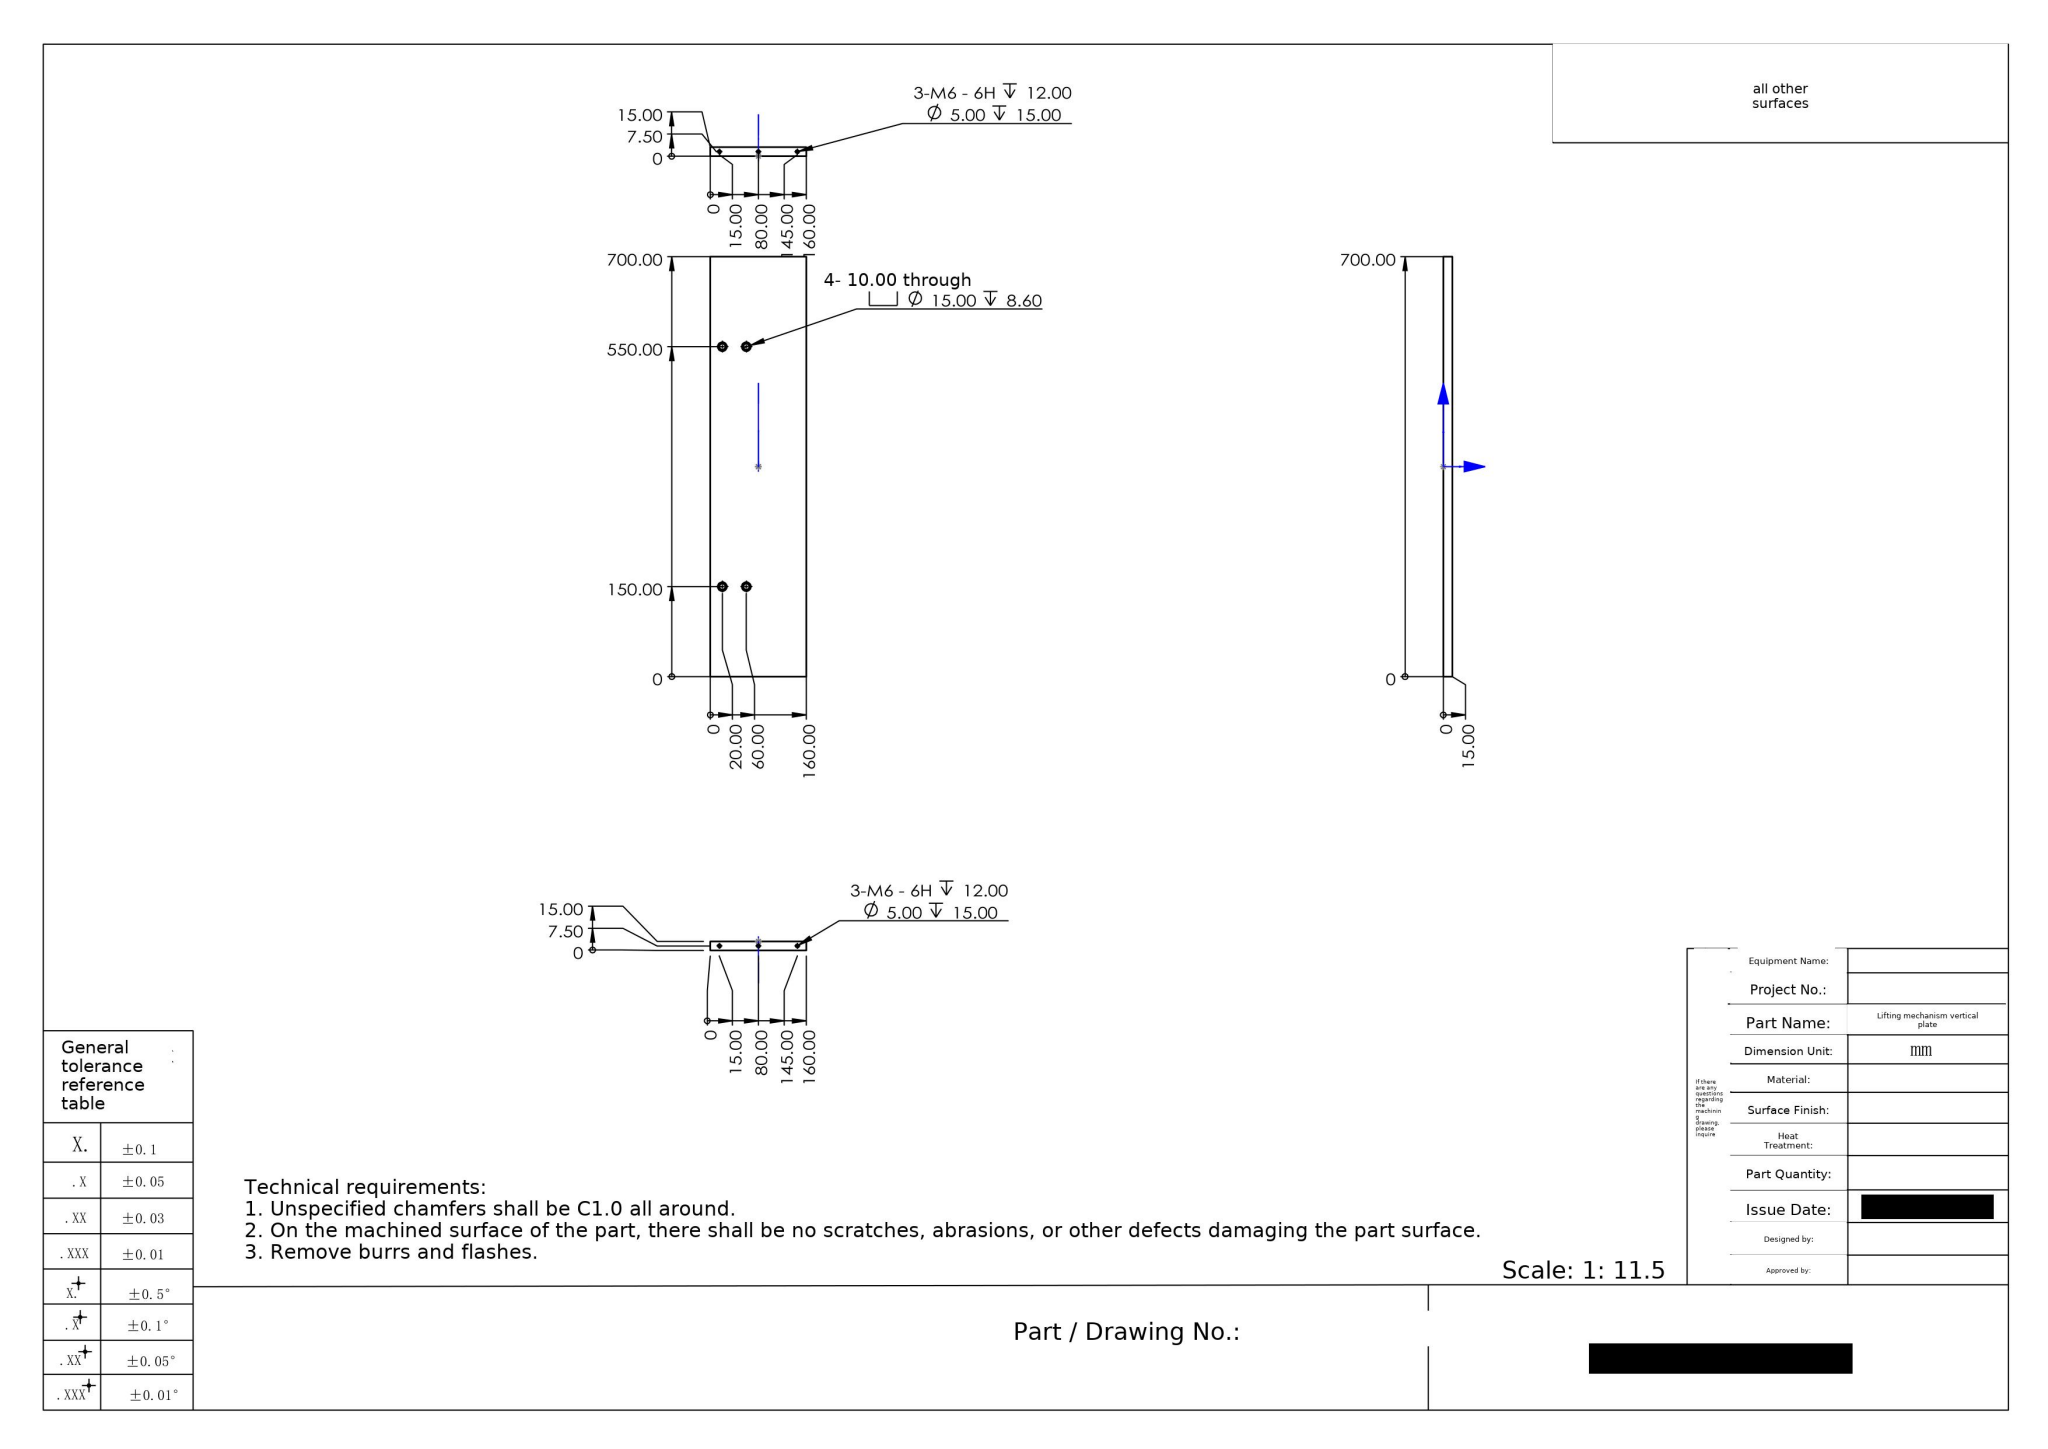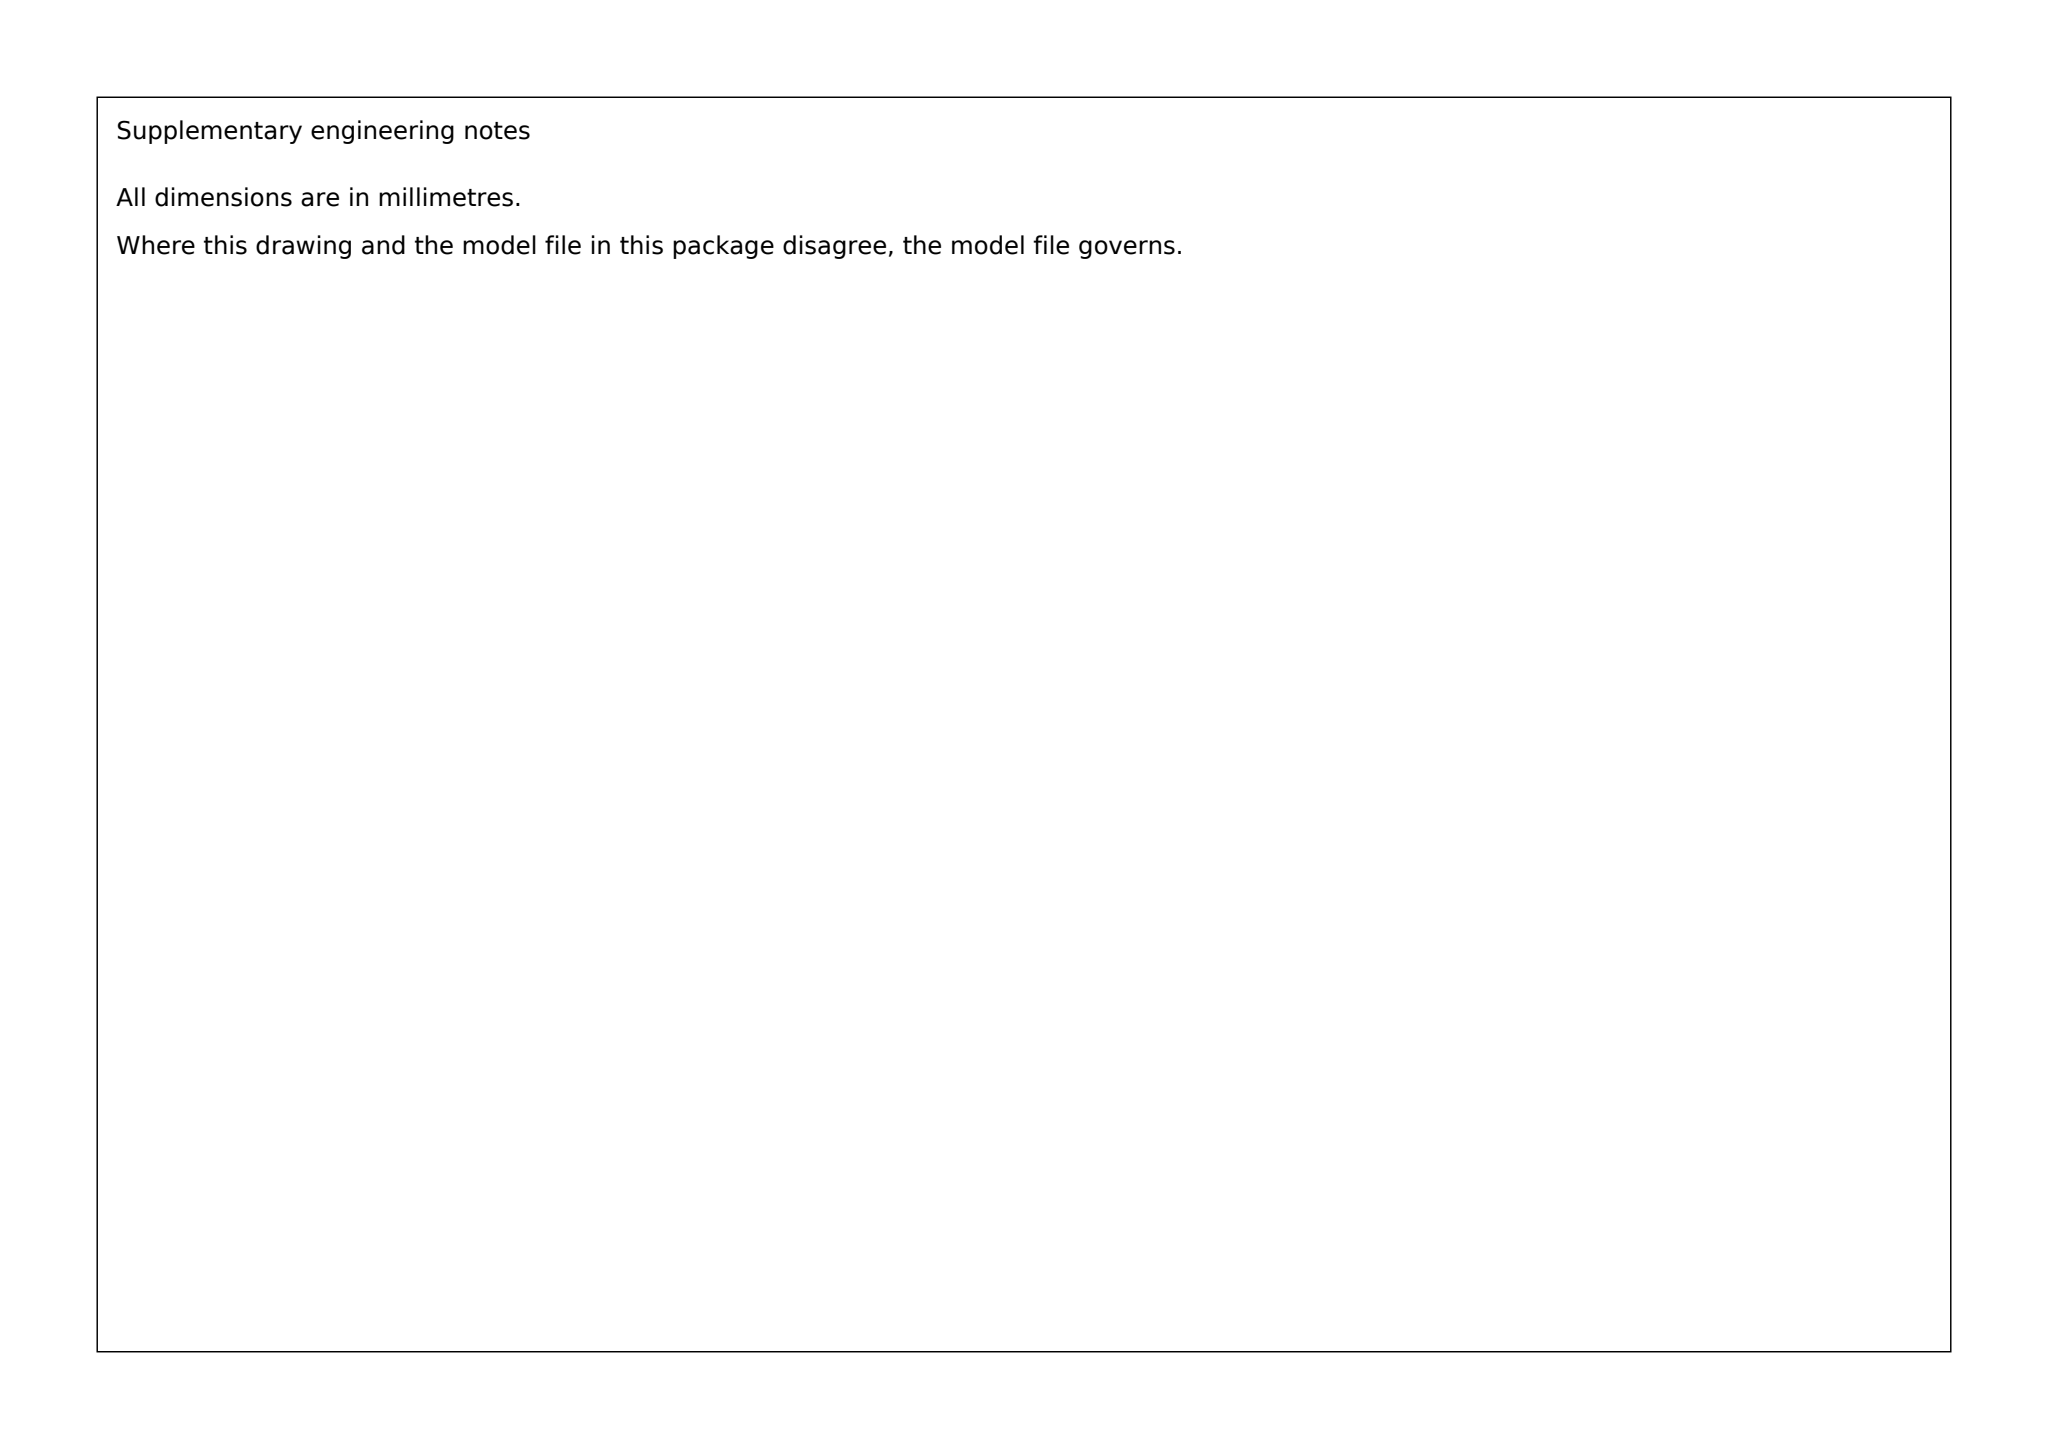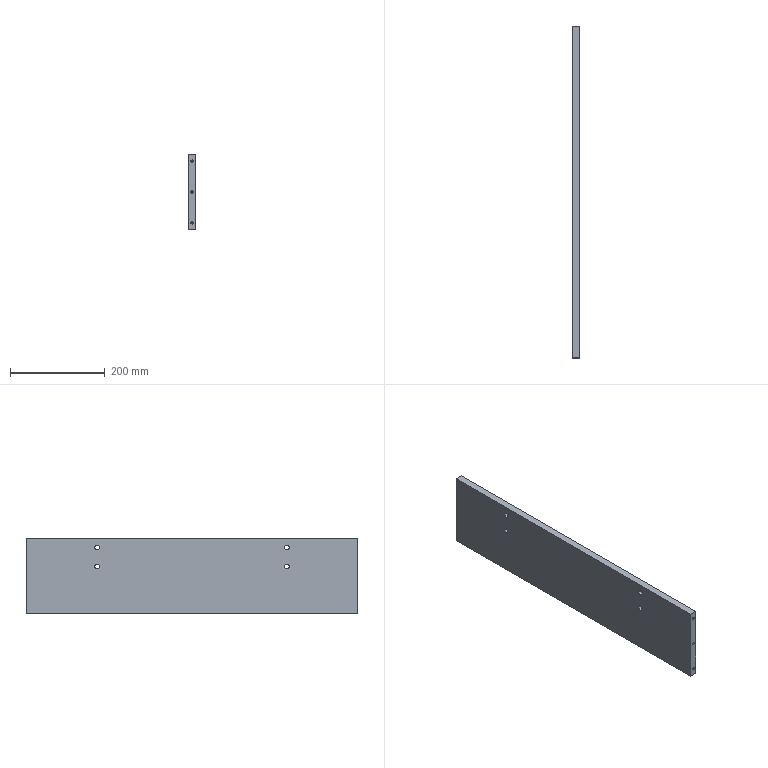Part | SolidWorks | mm | 1 solid | 50 faces | box 15 x 700 x 160 mm | volume 1670084 mm3 | cylinder 28 | cone 12 | plane 10 | commonest cylinder face diameters 5 x12 15 x8 10 x8
build123d program:
from build123d import *

# Parameters (mm, degrees)
SKETCH1_W                                       = 160
SKETCH1_H                                       = 700
BOSS_EXTRUDE1_DEPTH                             = 15
M8_HEX_SOCKET_HEAD_CAP_SCREW_CBORE1_D           = 10
M8_HEX_SOCKET_HEAD_CAP_SCREW_CBORE1_CBORE_D     = 15
M8_HEX_SOCKET_HEAD_CAP_SCREW_CBORE1_CBORE_DEPTH = 8.6
M6_TAPPED_HOLE1_AT_2_COUNT                      = 2
M6_TAPPED_HOLE1_AT_2_PITCH                      = 65
M6_TAPPED_HOLE1_AT_3_COUNT                      = 2
M6_TAPPED_HOLE1_AT_3_PITCH                      = 130


with BuildPart() as part:
    # Sketch1 → Boss-Extrude1 (new body)
    with BuildSketch(Plane(origin=(0, 0, 0), x_dir=(0, 0, -1), z_dir=(1, 0, 0))):
        Rectangle(SKETCH1_W, SKETCH1_H)
    extrude(amount=BOSS_EXTRUDE1_DEPTH)

    # M8 Hex Socket Head Cap Screw CBORE1 (through all)
    with Locations(Plane(origin=(15, 0, 0), x_dir=(0, 0, -1), z_dir=(1, 0, 0))):
        with Locations((-60, 200), (-20, 200), (-60, -200), (-20, -200)):
            CounterBoreHole(M8_HEX_SOCKET_HEAD_CAP_SCREW_CBORE1_D / 2, M8_HEX_SOCKET_HEAD_CAP_SCREW_CBORE1_CBORE_D / 2, M8_HEX_SOCKET_HEAD_CAP_SCREW_CBORE1_CBORE_DEPTH)

    # Sketch6 → M6 Tapped Hole1 (revolve, cut)
    with BuildSketch(Plane(origin=(7.5, 350, 65), x_dir=(0, 0, 1), z_dir=(1, 0, 0))):
        Polygon((0, 0), (0, 16.502), (2.5, 15), (2.5, 0), align=None)
    m6_tapped_hole1 = revolve(axis=Axis((7.5, 356.35, 65), (0, -1, 0)), mode=Mode.SUBTRACT)

    # M6 Tapped Hole1 at 2: M6 Tapped Hole1 ×2
    with Locations(*[(0, 0, -i * M6_TAPPED_HOLE1_AT_2_PITCH) for i in range(1, M6_TAPPED_HOLE1_AT_2_COUNT)]):
        add(m6_tapped_hole1, mode=Mode.SUBTRACT)

    # M6 Tapped Hole1 at 3: M6 Tapped Hole1 ×2
    with Locations(*[(0, 0, -i * M6_TAPPED_HOLE1_AT_3_PITCH) for i in range(1, M6_TAPPED_HOLE1_AT_3_COUNT)]):
        add(m6_tapped_hole1, mode=Mode.SUBTRACT)

    # Mirror1: M6 Tapped Hole1 across plane
    add(m6_tapped_hole1.mirror(Plane.ZX), mode=Mode.SUBTRACT)

    # Mirror1 copy 1 sketch → Mirror1 copy 1 (revolve, cut)
    with BuildSketch(Plane(origin=(7.5, -350, 0), x_dir=(0, 0, 1), z_dir=(1, 0, 0))):
        Polygon((0, 0), (0, -16.502), (2.5, -15), (2.5, 0), align=None)
    revolve(axis=Axis((7.5, -356.35, 0), (0, -1, 0)), mode=Mode.SUBTRACT)

    # Mirror1 copy 2 sketch → Mirror1 copy 2 (revolve, cut)
    with BuildSketch(Plane(origin=(7.5, -350, -65), x_dir=(0, 0, 1), z_dir=(1, 0, 0))):
        Polygon((0, 0), (0, -16.502), (2.5, -15), (2.5, 0), align=None)
    revolve(axis=Axis((7.5, -356.35, -65), (0, -1, 0)), mode=Mode.SUBTRACT)


solid = part.part